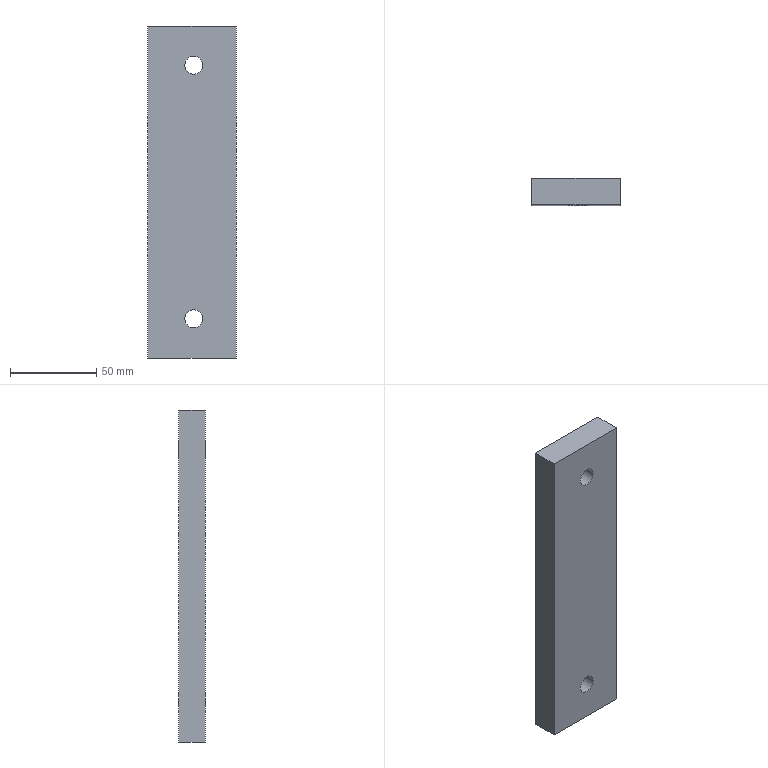Component | SolidWorks | Three-PhaseAsynchronousMotor-1_MotorMount-1 | 1 solid | 10 faces | box 51.1 x 15.4 x 192.5 mm | volume 148819 mm3 | plane 6 | cylinder 4 | commonest cylinder face diameters 10.5 x4
STEP:
#1=COLOUR_RGB('',0.7922,0.8196,0.9333);
#2=FILL_AREA_STYLE_COLOUR('',#1);
#3=FILL_AREA_STYLE('',(#2));
#4=SURFACE_STYLE_FILL_AREA(#3);
#5=SURFACE_SIDE_STYLE('',(#4));
#6=SURFACE_STYLE_USAGE(.BOTH.,#5);
#7=PRESENTATION_STYLE_ASSIGNMENT((#6));
#8=CARTESIAN_POINT('',(-15.872,-10.811,-0.1693));
#9=VERTEX_POINT('',#8);
#10=CARTESIAN_POINT('',(-16.285,-10.811,-0.1693));
#11=VERTEX_POINT('',#10);
#12=CARTESIAN_POINT('',(-16.079,-10.811,-0.1693));
#13=DIRECTION('',(0.,-1.,0.));
#14=DIRECTION('',(-1.,0.,0.));
#15=AXIS2_PLACEMENT_3D('',#12,#13,#14);
#16=CIRCLE('',#15,0.2067);
#17=EDGE_CURVE('',#9,#11,#16,.T.);
#18=ORIENTED_EDGE('',*,*,#17,.F.);
#19=CARTESIAN_POINT('',(-15.872,-11.417,-0.1693));
#20=VERTEX_POINT('',#19);
#21=CARTESIAN_POINT('',(-15.872,-10.811,-0.1693));
#22=DIRECTION('',(0.,-1.,0.));
#23=VECTOR('',#22,39.37);
#24=LINE('',#21,#23);
#25=EDGE_CURVE('',#9,#20,#24,.T.);
#26=ORIENTED_EDGE('',*,*,#25,.T.);
#27=CARTESIAN_POINT('',(-16.285,-11.417,-0.1693));
#28=VERTEX_POINT('',#27);
#29=CARTESIAN_POINT('',(-16.079,-11.417,-0.1693));
#30=DIRECTION('',(0.,-1.,0.));
#31=DIRECTION('',(-1.,0.,0.));
#32=AXIS2_PLACEMENT_3D('',#29,#30,#31);
#33=CIRCLE('',#32,0.2067);
#34=EDGE_CURVE('',#20,#28,#33,.T.);
#35=ORIENTED_EDGE('',*,*,#34,.T.);
#36=CARTESIAN_POINT('',(-16.285,-10.811,-0.1693));
#37=DIRECTION('',(0.,-1.,0.));
#38=VECTOR('',#37,39.37);
#39=LINE('',#36,#38);
#40=EDGE_CURVE('',#11,#28,#39,.T.);
#41=ORIENTED_EDGE('',*,*,#40,.F.);
#42=EDGE_LOOP('',(#18,#26,#35,#41));
#43=FACE_OUTER_BOUND('',#42,.T.);
#44=CARTESIAN_POINT('',(-16.079,-10.811,-0.1693));
#45=DIRECTION('',(0.,-1.,0.));
#46=DIRECTION('',(-1.,0.,0.));
#47=AXIS2_PLACEMENT_3D('',#44,#45,#46);
#48=CYLINDRICAL_SURFACE('',#47,0.2067);
#49=ADVANCED_FACE('',(#43),#48,.F.);
#50=CARTESIAN_POINT('',(-15.872,-10.811,-5.957));
#51=VERTEX_POINT('',#50);
#52=CARTESIAN_POINT('',(-16.285,-10.811,-5.957));
#53=VERTEX_POINT('',#52);
#54=CARTESIAN_POINT('',(-16.079,-10.811,-5.957));
#55=DIRECTION('',(0.,-1.,0.));
#56=DIRECTION('',(-1.,0.,0.));
#57=AXIS2_PLACEMENT_3D('',#54,#55,#56);
#58=CIRCLE('',#57,0.2067);
#59=EDGE_CURVE('',#51,#53,#58,.T.);
#60=ORIENTED_EDGE('',*,*,#59,.F.);
#61=CARTESIAN_POINT('',(-15.872,-11.417,-5.957));
#62=VERTEX_POINT('',#61);
#63=CARTESIAN_POINT('',(-15.872,-10.811,-5.957));
#64=DIRECTION('',(0.,-1.,0.));
#65=VECTOR('',#64,39.37);
#66=LINE('',#63,#65);
#67=EDGE_CURVE('',#51,#62,#66,.T.);
#68=ORIENTED_EDGE('',*,*,#67,.T.);
#69=CARTESIAN_POINT('',(-16.285,-11.417,-5.957));
#70=VERTEX_POINT('',#69);
#71=CARTESIAN_POINT('',(-16.079,-11.417,-5.957));
#72=DIRECTION('',(0.,-1.,0.));
#73=DIRECTION('',(-1.,0.,0.));
#74=AXIS2_PLACEMENT_3D('',#71,#72,#73);
#75=CIRCLE('',#74,0.2067);
#76=EDGE_CURVE('',#62,#70,#75,.T.);
#77=ORIENTED_EDGE('',*,*,#76,.T.);
#78=CARTESIAN_POINT('',(-16.285,-10.811,-5.957));
#79=DIRECTION('',(0.,-1.,0.));
#80=VECTOR('',#79,39.37);
#81=LINE('',#78,#80);
#82=EDGE_CURVE('',#53,#70,#81,.T.);
#83=ORIENTED_EDGE('',*,*,#82,.F.);
#84=EDGE_LOOP('',(#60,#68,#77,#83));
#85=FACE_OUTER_BOUND('',#84,.T.);
#86=CARTESIAN_POINT('',(-16.079,-10.811,-5.957));
#87=DIRECTION('',(0.,-1.,0.));
#88=DIRECTION('',(-1.,0.,0.));
#89=AXIS2_PLACEMENT_3D('',#86,#87,#88);
#90=CYLINDRICAL_SURFACE('',#89,0.2067);
#91=ADVANCED_FACE('',(#85),#90,.F.);
#92=CARTESIAN_POINT('',(-16.079,-11.417,-0.1693));
#93=DIRECTION('',(0.,-1.,0.));
#94=DIRECTION('',(-1.,0.,0.));
#95=AXIS2_PLACEMENT_3D('',#92,#93,#94);
#96=CIRCLE('',#95,0.2067);
#97=EDGE_CURVE('',#28,#20,#96,.T.);
#98=ORIENTED_EDGE('',*,*,#97,.F.);
#99=ORIENTED_EDGE('',*,*,#34,.F.);
#100=EDGE_LOOP('',(#98,#99));
#101=FACE_BOUND('',#100,.T.);
#102=CARTESIAN_POINT('',(-15.114,-11.417,0.7264));
#103=VERTEX_POINT('',#102);
#104=CARTESIAN_POINT('',(-15.114,-11.417,-6.852));
#105=VERTEX_POINT('',#104);
#106=CARTESIAN_POINT('',(-15.114,-11.417,-6.852));
#107=DIRECTION('',(0.,0.,-1.));
#108=VECTOR('',#107,39.37);
#109=LINE('',#106,#108);
#110=EDGE_CURVE('',#103,#105,#109,.T.);
#111=ORIENTED_EDGE('',*,*,#110,.F.);
#112=CARTESIAN_POINT('',(-17.126,-11.417,0.7264));
#113=VERTEX_POINT('',#112);
#114=CARTESIAN_POINT('',(-17.126,-11.417,0.7264));
#115=DIRECTION('',(1.,0.,0.));
#116=VECTOR('',#115,39.37);
#117=LINE('',#114,#116);
#118=EDGE_CURVE('',#113,#103,#117,.T.);
#119=ORIENTED_EDGE('',*,*,#118,.F.);
#120=CARTESIAN_POINT('',(-17.126,-11.417,-6.852));
#121=VERTEX_POINT('',#120);
#122=CARTESIAN_POINT('',(-17.126,-11.417,-6.852));
#123=DIRECTION('',(0.,0.,1.));
#124=VECTOR('',#123,39.37);
#125=LINE('',#122,#124);
#126=EDGE_CURVE('',#121,#113,#125,.T.);
#127=ORIENTED_EDGE('',*,*,#126,.F.);
#128=CARTESIAN_POINT('',(-17.126,-11.417,-6.852));
#129=DIRECTION('',(-1.,0.,0.));
#130=VECTOR('',#129,39.37);
#131=LINE('',#128,#130);
#132=EDGE_CURVE('',#105,#121,#131,.T.);
#133=ORIENTED_EDGE('',*,*,#132,.F.);
#134=EDGE_LOOP('',(#111,#119,#127,#133));
#135=FACE_OUTER_BOUND('',#134,.T.);
#136=CARTESIAN_POINT('',(-16.079,-11.417,-5.957));
#137=DIRECTION('',(0.,-1.,0.));
#138=DIRECTION('',(-1.,0.,0.));
#139=AXIS2_PLACEMENT_3D('',#136,#137,#138);
#140=CIRCLE('',#139,0.2067);
#141=EDGE_CURVE('',#70,#62,#140,.T.);
#142=ORIENTED_EDGE('',*,*,#141,.F.);
#143=ORIENTED_EDGE('',*,*,#76,.F.);
#144=EDGE_LOOP('',(#142,#143));
#145=FACE_BOUND('',#144,.T.);
#146=CARTESIAN_POINT('',(-17.126,-11.417,-6.852));
#147=DIRECTION('',(0.,1.,0.));
#148=DIRECTION('',(1.,0.,0.));
#149=AXIS2_PLACEMENT_3D('',#146,#147,#148);
#150=PLANE('',#149);
#151=ADVANCED_FACE('',(#101,#135,#145),#150,.F.);
#152=ORIENTED_EDGE('',*,*,#25,.F.);
#153=CARTESIAN_POINT('',(-16.079,-10.811,-0.1693));
#154=DIRECTION('',(0.,-1.,0.));
#155=DIRECTION('',(-1.,0.,0.));
#156=AXIS2_PLACEMENT_3D('',#153,#154,#155);
#157=CIRCLE('',#156,0.2067);
#158=EDGE_CURVE('',#11,#9,#157,.T.);
#159=ORIENTED_EDGE('',*,*,#158,.F.);
#160=ORIENTED_EDGE('',*,*,#40,.T.);
#161=ORIENTED_EDGE('',*,*,#97,.T.);
#162=EDGE_LOOP('',(#152,#159,#160,#161));
#163=FACE_OUTER_BOUND('',#162,.T.);
#164=CARTESIAN_POINT('',(-16.079,-10.811,-0.1693));
#165=DIRECTION('',(0.,-1.,0.));
#166=DIRECTION('',(-1.,0.,0.));
#167=AXIS2_PLACEMENT_3D('',#164,#165,#166);
#168=CYLINDRICAL_SURFACE('',#167,0.2067);
#169=ADVANCED_FACE('',(#163),#168,.F.);
#170=CARTESIAN_POINT('',(-15.114,-10.811,-6.852));
#171=VERTEX_POINT('',#170);
#172=CARTESIAN_POINT('',(-17.126,-10.811,-6.852));
#173=VERTEX_POINT('',#172);
#174=CARTESIAN_POINT('',(-17.126,-10.811,-6.852));
#175=DIRECTION('',(-1.,0.,0.));
#176=VECTOR('',#175,39.37);
#177=LINE('',#174,#176);
#178=EDGE_CURVE('',#171,#173,#177,.T.);
#179=ORIENTED_EDGE('',*,*,#178,.F.);
#180=CARTESIAN_POINT('',(-15.114,-10.811,-6.852));
#181=DIRECTION('',(0.,1.,0.));
#182=VECTOR('',#181,39.37);
#183=LINE('',#180,#182);
#184=EDGE_CURVE('',#105,#171,#183,.T.);
#185=ORIENTED_EDGE('',*,*,#184,.F.);
#186=ORIENTED_EDGE('',*,*,#132,.T.);
#187=CARTESIAN_POINT('',(-17.126,-10.811,-6.852));
#188=DIRECTION('',(0.,-1.,0.));
#189=VECTOR('',#188,39.37);
#190=LINE('',#187,#189);
#191=EDGE_CURVE('',#173,#121,#190,.T.);
#192=ORIENTED_EDGE('',*,*,#191,.F.);
#193=EDGE_LOOP('',(#179,#185,#186,#192));
#194=FACE_OUTER_BOUND('',#193,.T.);
#195=CARTESIAN_POINT('',(-17.126,-10.811,-6.852));
#196=DIRECTION('',(0.,0.,1.));
#197=DIRECTION('',(1.,0.,0.));
#198=AXIS2_PLACEMENT_3D('',#195,#196,#197);
#199=PLANE('',#198);
#200=ADVANCED_FACE('',(#194),#199,.F.);
#201=CARTESIAN_POINT('',(-15.114,-10.811,0.7264));
#202=VERTEX_POINT('',#201);
#203=CARTESIAN_POINT('',(-15.114,-10.811,-6.852));
#204=DIRECTION('',(0.,0.,-1.));
#205=VECTOR('',#204,39.37);
#206=LINE('',#203,#205);
#207=EDGE_CURVE('',#202,#171,#206,.T.);
#208=ORIENTED_EDGE('',*,*,#207,.F.);
#209=CARTESIAN_POINT('',(-15.114,-10.811,0.7264));
#210=DIRECTION('',(0.,1.,0.));
#211=VECTOR('',#210,39.37);
#212=LINE('',#209,#211);
#213=EDGE_CURVE('',#103,#202,#212,.T.);
#214=ORIENTED_EDGE('',*,*,#213,.F.);
#215=ORIENTED_EDGE('',*,*,#110,.T.);
#216=ORIENTED_EDGE('',*,*,#184,.T.);
#217=EDGE_LOOP('',(#208,#214,#215,#216));
#218=FACE_OUTER_BOUND('',#217,.T.);
#219=CARTESIAN_POINT('',(-15.114,-10.811,-6.852));
#220=DIRECTION('',(-1.,0.,0.));
#221=DIRECTION('',(0.,0.,1.));
#222=AXIS2_PLACEMENT_3D('',#219,#220,#221);
#223=PLANE('',#222);
#224=ADVANCED_FACE('',(#218),#223,.F.);
#225=CARTESIAN_POINT('',(-17.126,-10.811,0.7264));
#226=VERTEX_POINT('',#225);
#227=CARTESIAN_POINT('',(-17.126,-10.811,0.7264));
#228=DIRECTION('',(1.,0.,0.));
#229=VECTOR('',#228,39.37);
#230=LINE('',#227,#229);
#231=EDGE_CURVE('',#226,#202,#230,.T.);
#232=ORIENTED_EDGE('',*,*,#231,.F.);
#233=CARTESIAN_POINT('',(-17.126,-10.811,0.7264));
#234=DIRECTION('',(0.,1.,0.));
#235=VECTOR('',#234,39.37);
#236=LINE('',#233,#235);
#237=EDGE_CURVE('',#113,#226,#236,.T.);
#238=ORIENTED_EDGE('',*,*,#237,.F.);
#239=ORIENTED_EDGE('',*,*,#118,.T.);
#240=ORIENTED_EDGE('',*,*,#213,.T.);
#241=EDGE_LOOP('',(#232,#238,#239,#240));
#242=FACE_OUTER_BOUND('',#241,.T.);
#243=CARTESIAN_POINT('',(-17.126,-10.811,0.7264));
#244=DIRECTION('',(0.,0.,-1.));
#245=DIRECTION('',(-1.,0.,-0.));
#246=AXIS2_PLACEMENT_3D('',#243,#244,#245);
#247=PLANE('',#246);
#248=ADVANCED_FACE('',(#242),#247,.F.);
#249=CARTESIAN_POINT('',(-17.126,-10.811,-6.852));
#250=DIRECTION('',(0.,0.,1.));
#251=VECTOR('',#250,39.37);
#252=LINE('',#249,#251);
#253=EDGE_CURVE('',#173,#226,#252,.T.);
#254=ORIENTED_EDGE('',*,*,#253,.F.);
#255=ORIENTED_EDGE('',*,*,#191,.T.);
#256=ORIENTED_EDGE('',*,*,#126,.T.);
#257=ORIENTED_EDGE('',*,*,#237,.T.);
#258=EDGE_LOOP('',(#254,#255,#256,#257));
#259=FACE_OUTER_BOUND('',#258,.T.);
#260=CARTESIAN_POINT('',(-17.126,-10.811,-6.852));
#261=DIRECTION('',(1.,0.,0.));
#262=DIRECTION('',(0.,0.,-1.));
#263=AXIS2_PLACEMENT_3D('',#260,#261,#262);
#264=PLANE('',#263);
#265=ADVANCED_FACE('',(#259),#264,.F.);
#266=ORIENTED_EDGE('',*,*,#67,.F.);
#267=CARTESIAN_POINT('',(-16.079,-10.811,-5.957));
#268=DIRECTION('',(0.,-1.,0.));
#269=DIRECTION('',(-1.,0.,0.));
#270=AXIS2_PLACEMENT_3D('',#267,#268,#269);
#271=CIRCLE('',#270,0.2067);
#272=EDGE_CURVE('',#53,#51,#271,.T.);
#273=ORIENTED_EDGE('',*,*,#272,.F.);
#274=ORIENTED_EDGE('',*,*,#82,.T.);
#275=ORIENTED_EDGE('',*,*,#141,.T.);
#276=EDGE_LOOP('',(#266,#273,#274,#275));
#277=FACE_OUTER_BOUND('',#276,.T.);
#278=CARTESIAN_POINT('',(-16.079,-10.811,-5.957));
#279=DIRECTION('',(0.,-1.,0.));
#280=DIRECTION('',(-1.,0.,0.));
#281=AXIS2_PLACEMENT_3D('',#278,#279,#280);
#282=CYLINDRICAL_SURFACE('',#281,0.2067);
#283=ADVANCED_FACE('',(#277),#282,.F.);
#284=ORIENTED_EDGE('',*,*,#158,.T.);
#285=ORIENTED_EDGE('',*,*,#17,.T.);
#286=EDGE_LOOP('',(#284,#285));
#287=FACE_BOUND('',#286,.T.);
#288=ORIENTED_EDGE('',*,*,#253,.T.);
#289=ORIENTED_EDGE('',*,*,#231,.T.);
#290=ORIENTED_EDGE('',*,*,#207,.T.);
#291=ORIENTED_EDGE('',*,*,#178,.T.);
#292=EDGE_LOOP('',(#288,#289,#290,#291));
#293=FACE_OUTER_BOUND('',#292,.T.);
#294=ORIENTED_EDGE('',*,*,#272,.T.);
#295=ORIENTED_EDGE('',*,*,#59,.T.);
#296=EDGE_LOOP('',(#294,#295));
#297=FACE_BOUND('',#296,.T.);
#298=CARTESIAN_POINT('',(-17.126,-10.811,-6.852));
#299=DIRECTION('',(0.,1.,0.));
#300=DIRECTION('',(1.,0.,0.));
#301=AXIS2_PLACEMENT_3D('',#298,#299,#300);
#302=PLANE('',#301);
#303=ADVANCED_FACE('',(#287,#293,#297),#302,.T.);
#304=CLOSED_SHELL('',(#49,#91,#151,#169,#200,#224,#248,#265,#283,#303));
#305=MANIFOLD_SOLID_BREP('',#304);
#306=STYLED_ITEM('',(#7),#305);
#307=(LENGTH_UNIT()NAMED_UNIT(*)SI_UNIT($,.METRE.));
#308=LENGTH_MEASURE_WITH_UNIT(LENGTH_MEASURE(0.0254),#307);
#309=DIMENSIONAL_EXPONENTS(1.,0.,0.,0.,0.,0.,0.);
#310=(CONVERSION_BASED_UNIT('',#308)LENGTH_UNIT()NAMED_UNIT(#309));
#311=UNCERTAINTY_MEASURE_WITH_UNIT(LENGTH_MEASURE(0.00001),#310,'','');
#312=(NAMED_UNIT(*)PLANE_ANGLE_UNIT()SI_UNIT($,.RADIAN.));
#313=(NAMED_UNIT(*)SI_UNIT($,.STERADIAN.)SOLID_ANGLE_UNIT());
#314=(GEOMETRIC_REPRESENTATION_CONTEXT(3)GLOBAL_UNCERTAINTY_ASSIGNED_CONTEXT((#311))GLOBAL_UNIT_ASSIGNED_CONTEXT((#310,#312,#313))REPRESENTATION_CONTEXT('',''));
#315=MECHANICAL_DESIGN_GEOMETRIC_PRESENTATION_REPRESENTATION('',(#306),#314);
#316=PRESENTATION_LAYER_ASSIGNMENT('','',(#306));
#317=CARTESIAN_POINT('',(0.,0.,0.));
#318=DIRECTION('',(0.,0.,1.));
#319=DIRECTION('',(1.,0.,0.));
#320=AXIS2_PLACEMENT_3D('',#317,#318,#319);
#321=(LENGTH_UNIT()NAMED_UNIT(*)SI_UNIT($,.METRE.));
#322=LENGTH_MEASURE_WITH_UNIT(LENGTH_MEASURE(0.0254),#321);
#323=DIMENSIONAL_EXPONENTS(1.,0.,0.,0.,0.,0.,0.);
#324=(CONVERSION_BASED_UNIT('',#322)LENGTH_UNIT()NAMED_UNIT(#323));
#325=UNCERTAINTY_MEASURE_WITH_UNIT(LENGTH_MEASURE(0.00001),#324,'','');
#326=(NAMED_UNIT(*)PLANE_ANGLE_UNIT()SI_UNIT($,.RADIAN.));
#327=(NAMED_UNIT(*)SI_UNIT($,.STERADIAN.)SOLID_ANGLE_UNIT());
#328=(GEOMETRIC_REPRESENTATION_CONTEXT(3)GLOBAL_UNCERTAINTY_ASSIGNED_CONTEXT((#325))GLOBAL_UNIT_ASSIGNED_CONTEXT((#324,#326,#327))REPRESENTATION_CONTEXT('',''));
#329=ADVANCED_BREP_SHAPE_REPRESENTATION('',(#305,#320),#328);